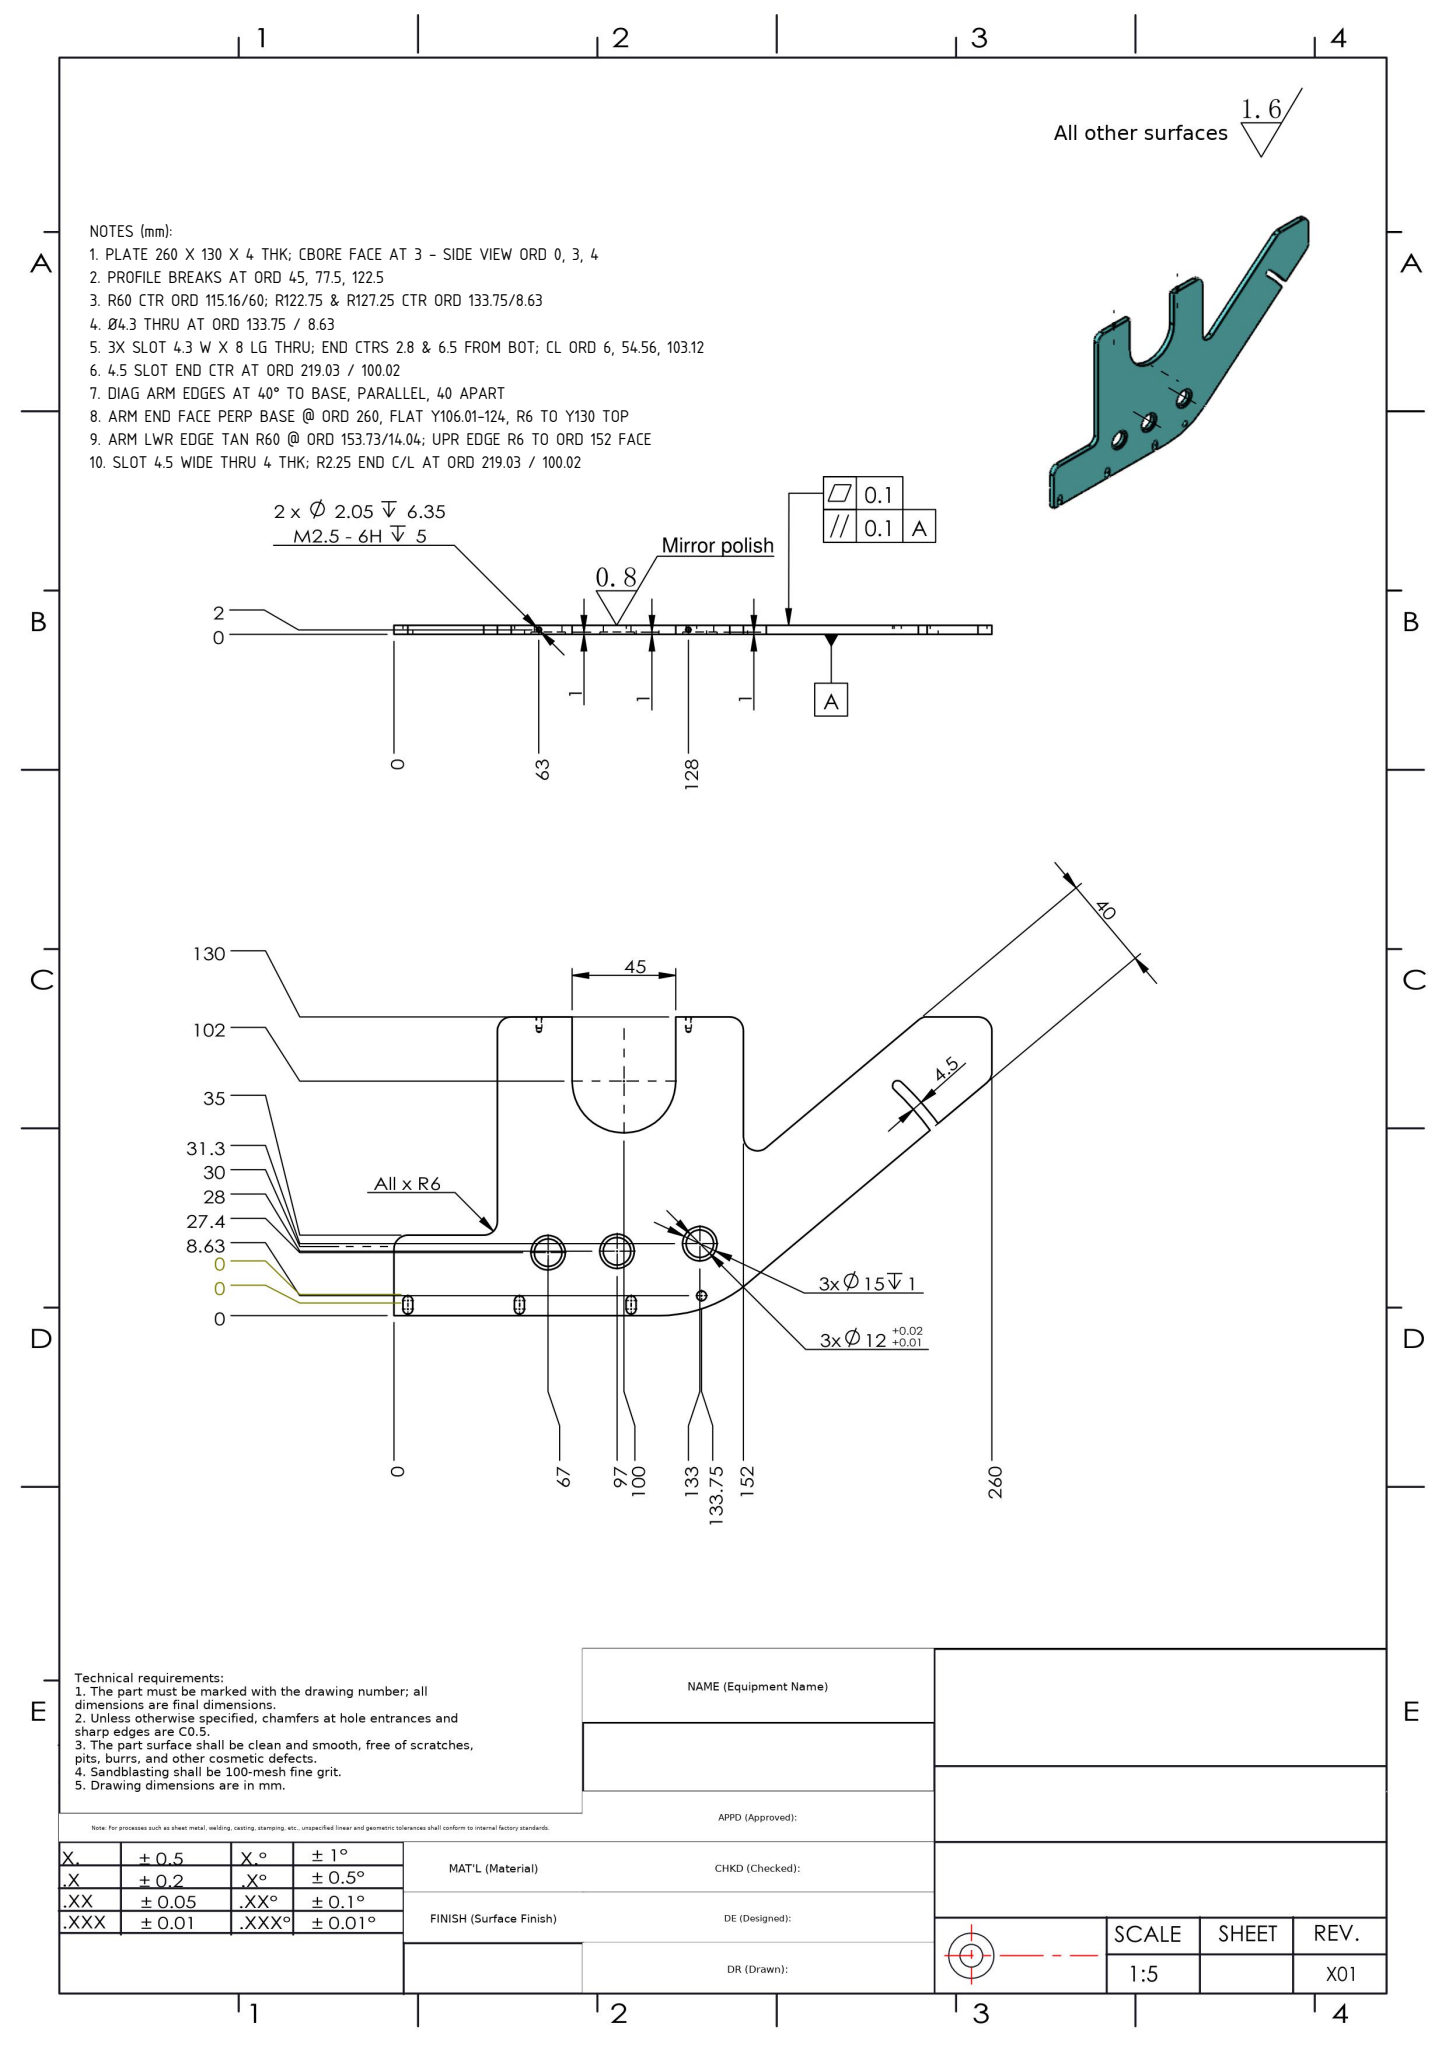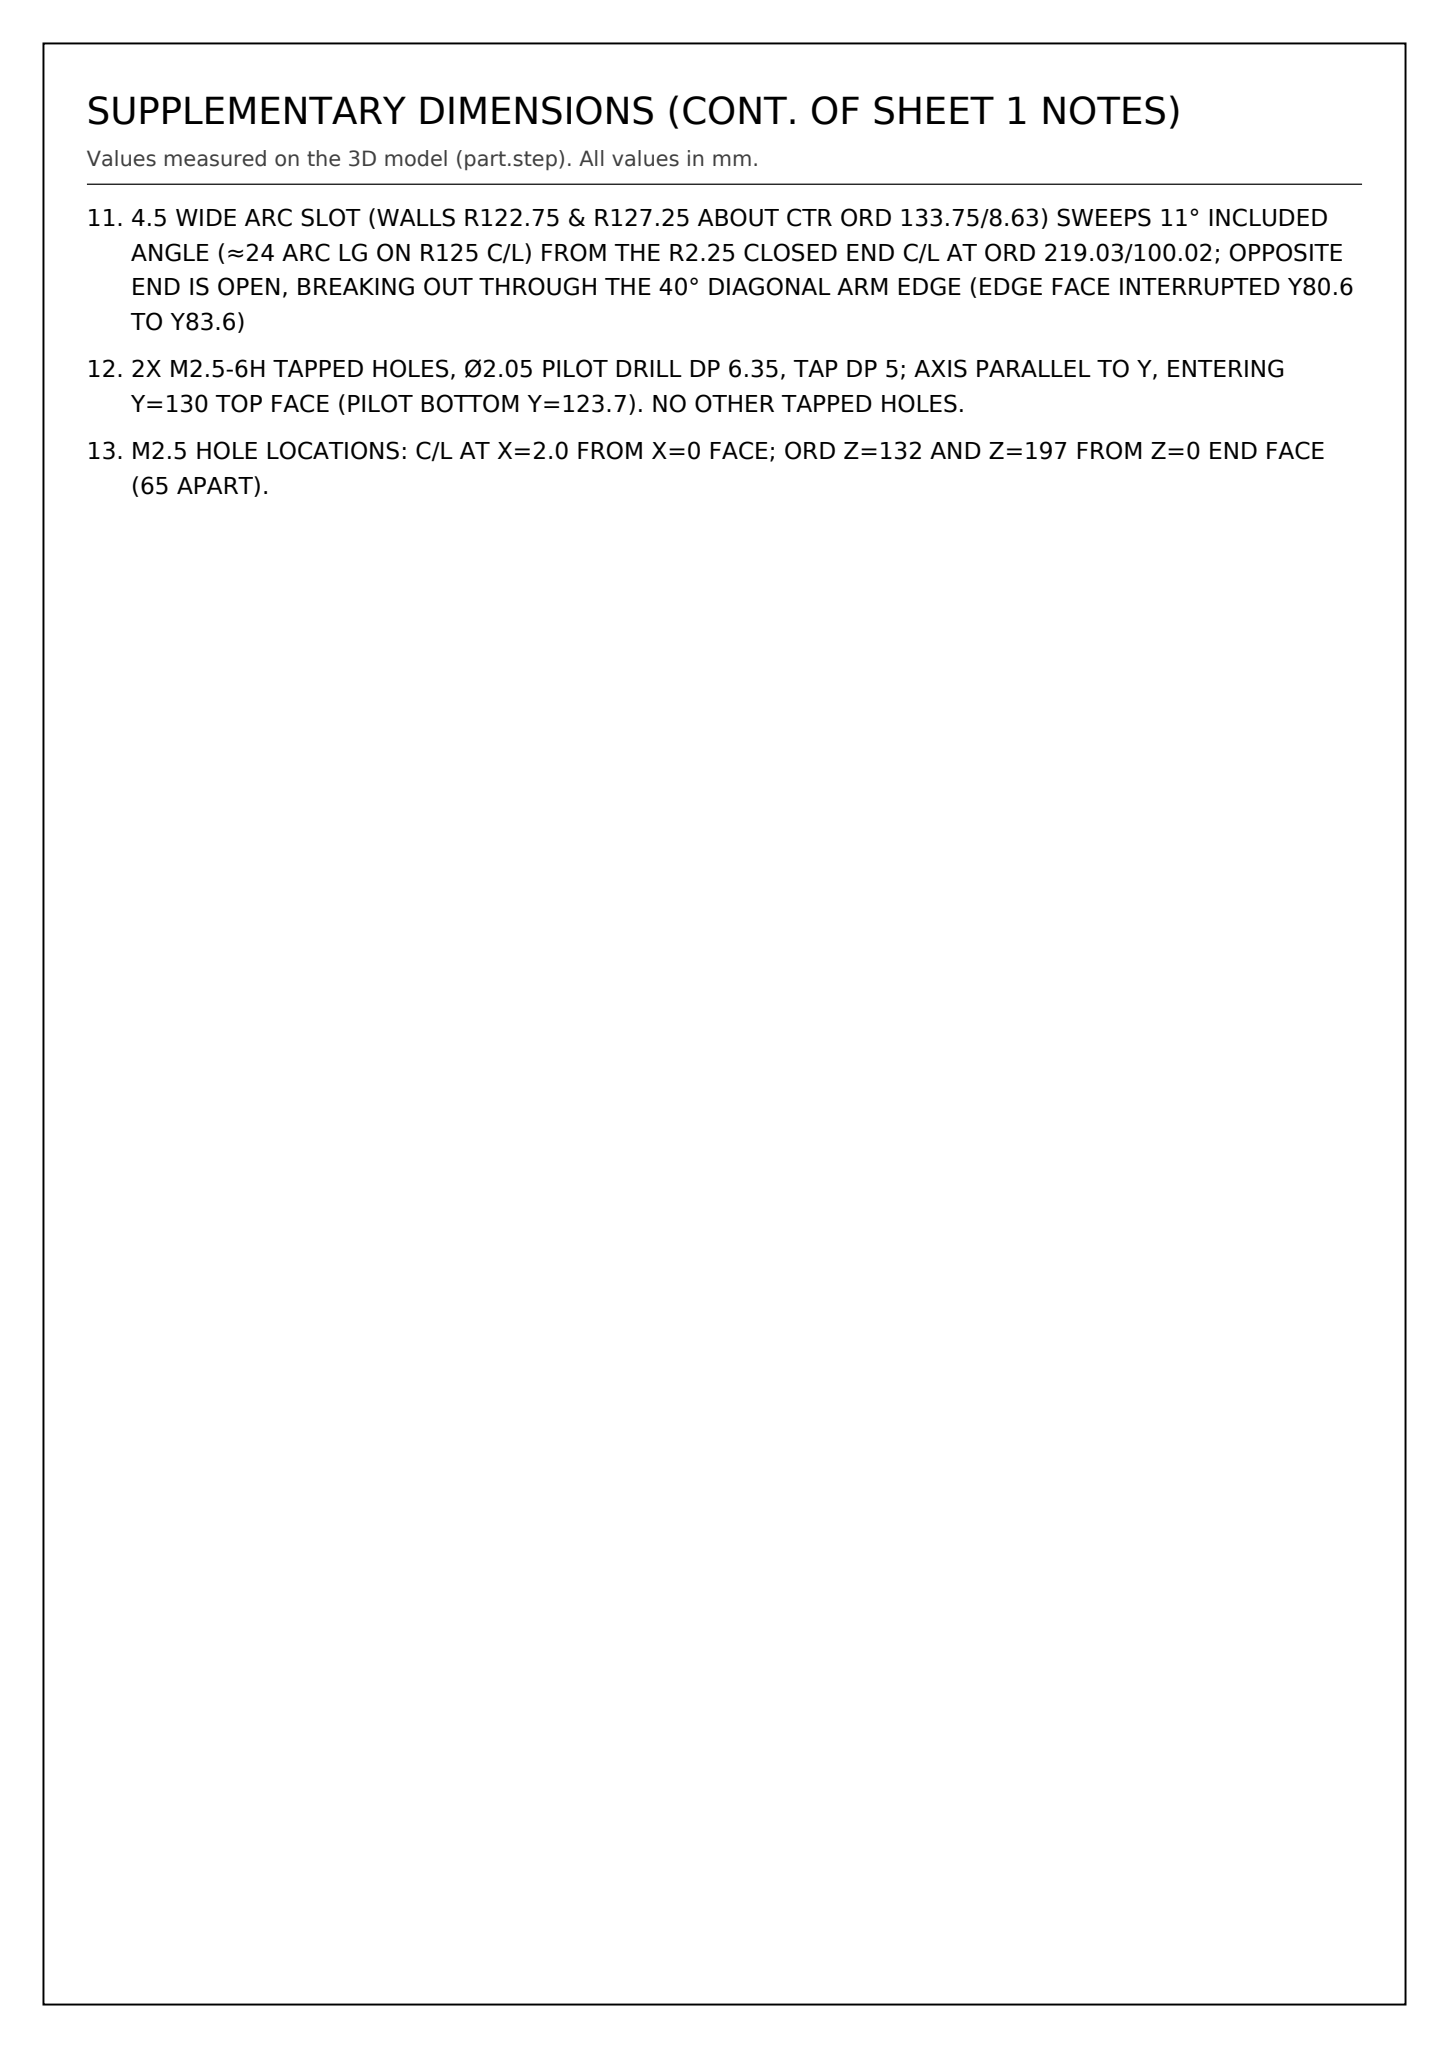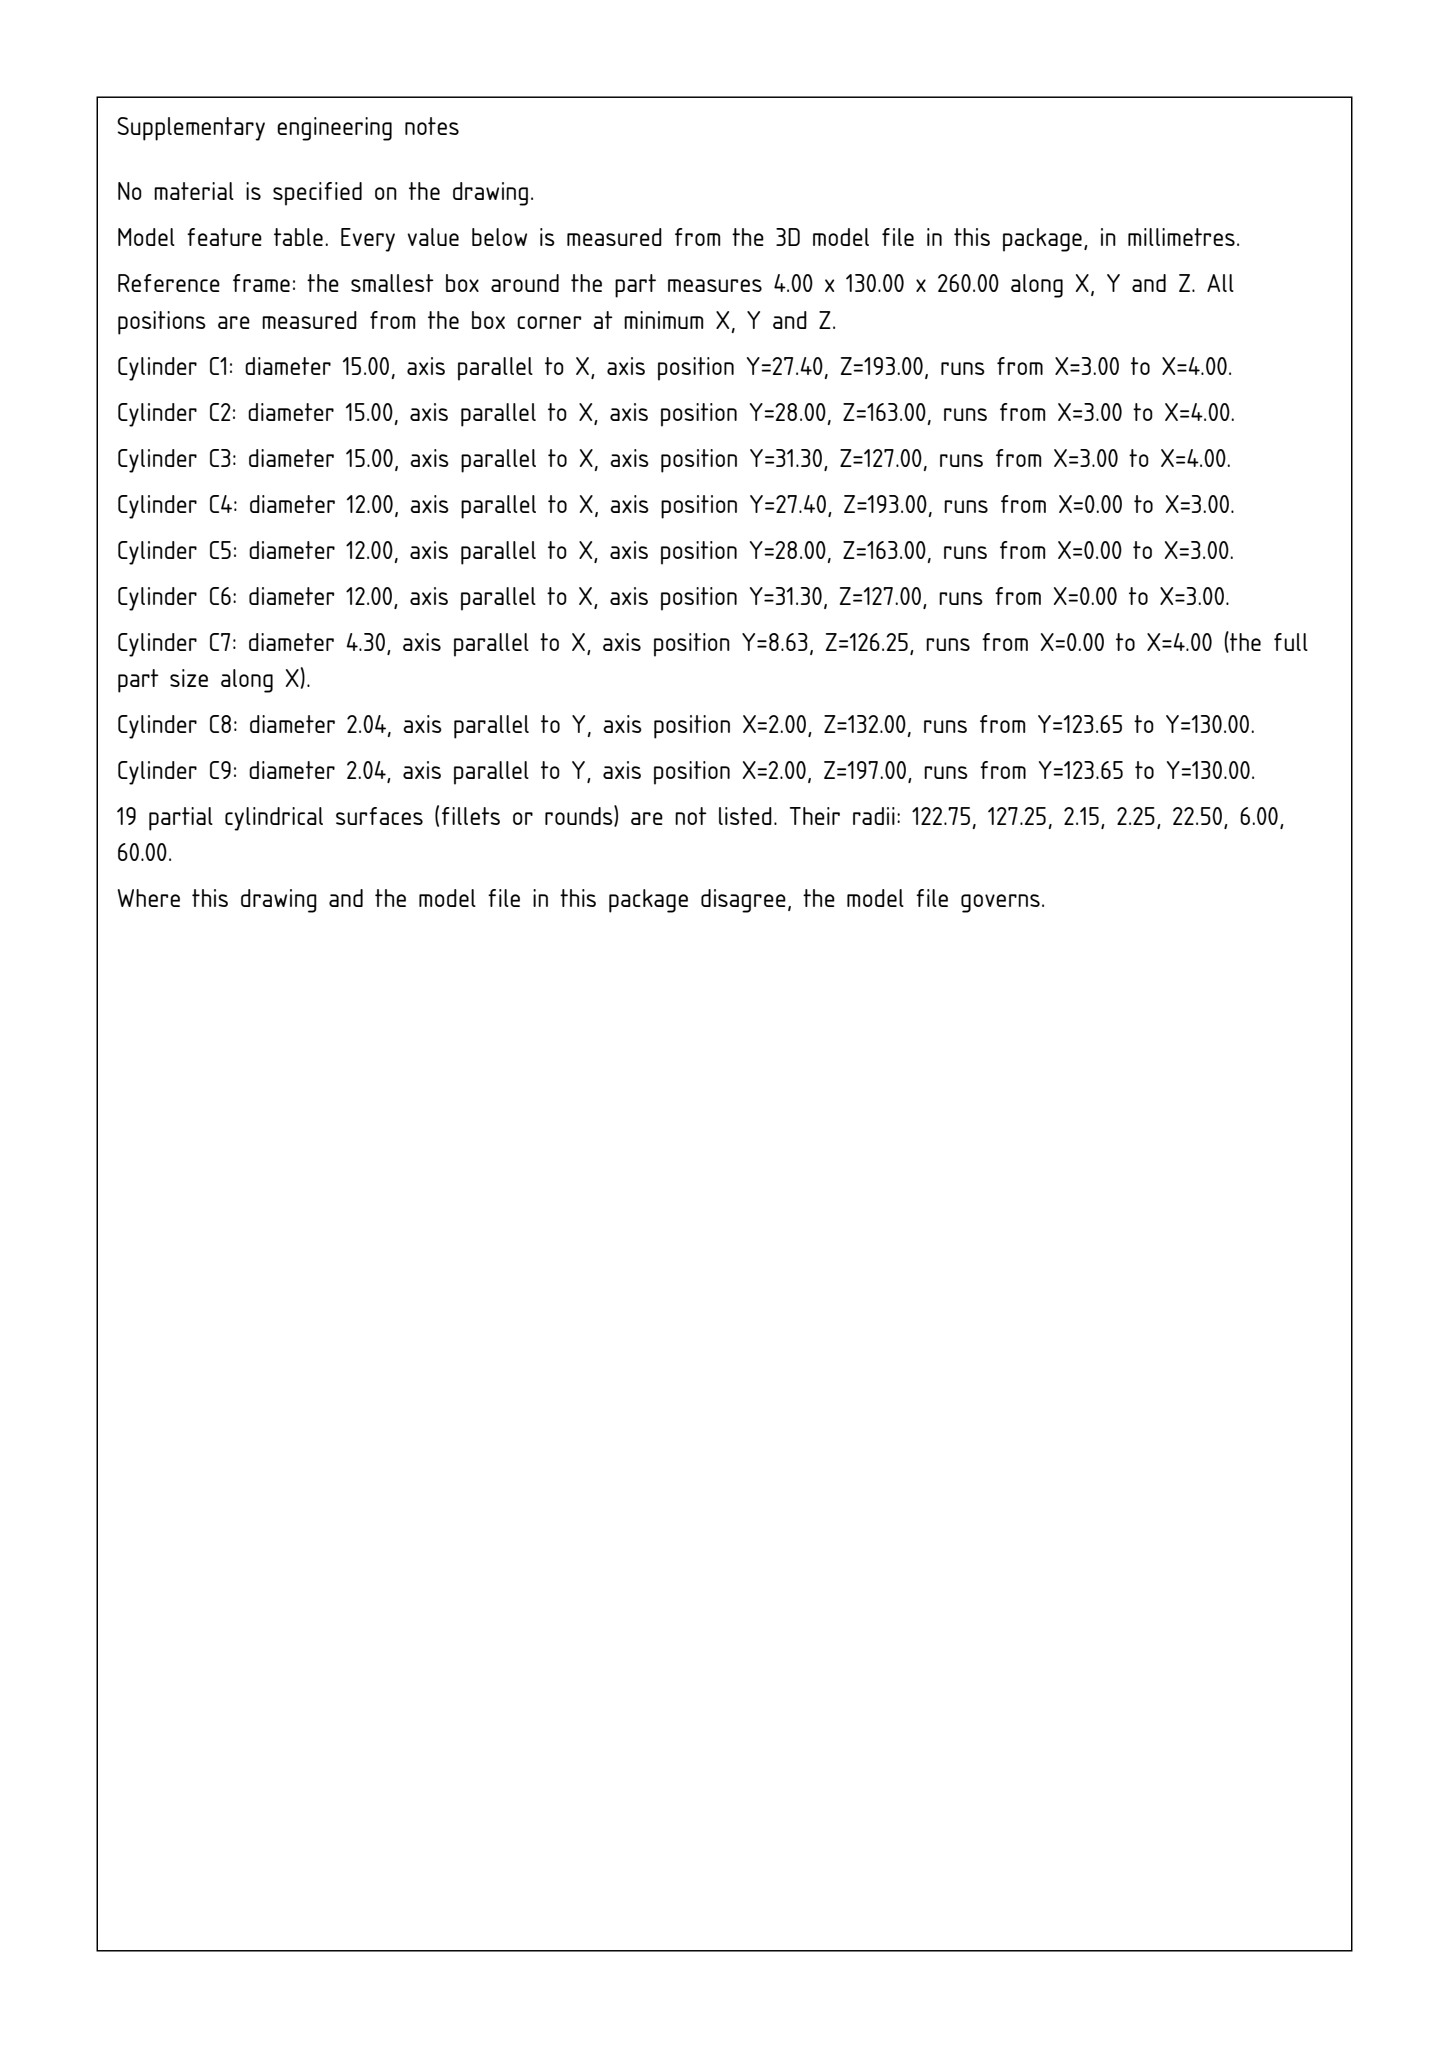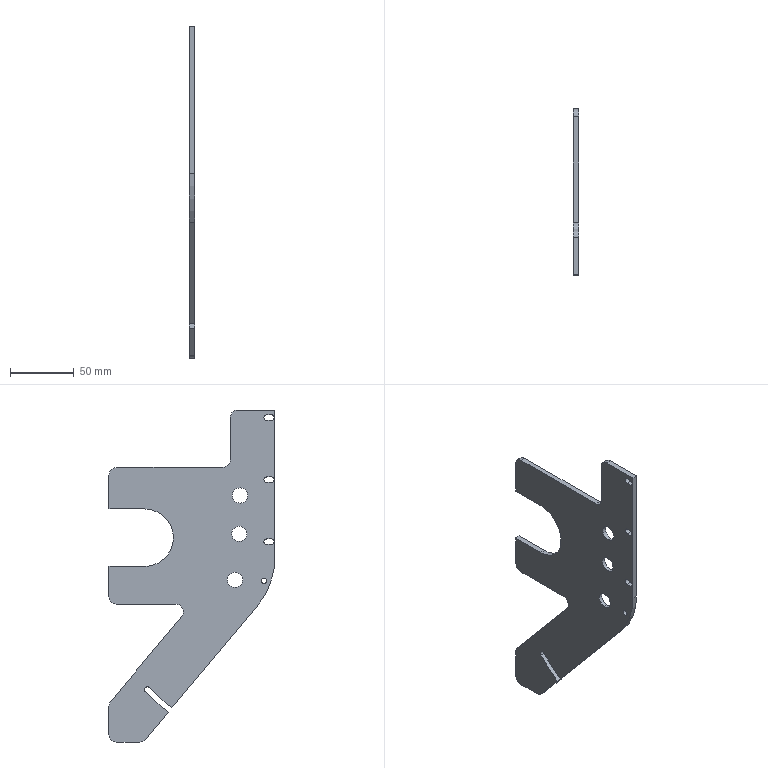Part | SolidWorks | mm | 1 solid | 66 faces | box 4 x 130 x 260 mm | volume 71713 mm3 | cylinder 37 | plane 25 | cone 4 | commonest cylinder face diameters 12 x14 4.3 x8 15 x6 2.05 x4 120 x1 245.5 x1 254.5 x1 4.5 x1
Drawing notes:
PLATE 260 X 130 X 4 THK; CBORE FACE AT 3 - SIDE VIEW ORD 0, 3, 4 | from the solid: bbox_xyz [4,130,260]; axis_planes x=0.0, 3.0 (3), 4.0
PROFILE BREAKS AT ORD 45, 77.5, 122.5 | from the solid: axis_planes z=215, 182.5, 137.5; ord = 260 - z
R60 CTR ORD 115.16/60; R122.75 & R127.25 CTR ORD 133.75/8.63 | from the solid: Ø120 at [y=60,z=144.84]; Ø245.5 & Ø254.5 at [y=8.63,z=126.25]
Ø4.3 THRU AT ORD 133.75 / 8.63 | from the solid: [4.3,"x",[null,8.63,126.25],4.0]; ord = 260-126.25 = 133.75
3X SLOT 4.3 W X 8 LG THRU; END CTRS 2.8 & 6.5 FROM BOT; CL ORD 6, 54.56, 103.12 | from the solid: Ø4.3 x-axis cyls at y=2.8 & 6.5, len 4.0 thru, z=156.88/205.44/254.0; 6.5-2.8+4.3=8; ord = 260-z
4.5 SLOT END CTR AT ORD 219.03 / 100.02 | from the solid: [4.5,"x",[null,100.02,40.97],4.0]; ord = 260-40.97 = 219.03
DIAG ARM EDGES AT 40° TO BASE, PARALLEL, 40 APART | from the solid: Upper edge tangent to R6 fillet ctr (ORD 231.88,Y124), lower edge tangent to R6 fillet ctr (ORD 254,Y106.01); common normal gives 40.0° to ORD axis and 40.00 perpendicular spacing (matches 40 width dim)
ARM END FACE PERP BASE @ ORD 260, FLAT Y106.01-124, R6 TO Y130 TOP | from the solid: Planar face normal z at z=0 (ORD 260 = 260-z); R6 (Ø12) fillet ctrs at y=106.01/z=6 and y=124/z=6; plane y=130 top face tangent to R6 ctr y=124, z=28.12 (ORD 231.88-254)
ARM LWR EDGE TAN R60 @ ORD 153.73/14.04; UPR EDGE R6 TO ORD 152 FACE | from the solid: Ø120 (R60) cyl ctr y=60,z=144.84 (ORD 115.16); dist from ctr to lower edge line = 59.99; R6 fillet ctr y=77.67,z=102 (ORD 158) tangent to upper edge and to plane z=108 (ORD 152)
SLOT 4.5 WIDE THRU 4 THK; R2.25 END C/L AT ORD 219.03 / 100.02 | from the solid: cylinders: [4.5,"x",[null,100.02,40.97],4.0,1]; bbox z=260 so ORD = 260-40.97 = 219.03; plate thk 4 (x planes 0.0 and 4.0)
4.5 WIDE ARC SLOT (WALLS R122.75 & R127.25 ABOUT CTR ORD 133.75/8.63) SWEEPS 11° INCLUDED ANGLE (≈24 ARC LG ON R125 C/L) FROM THE R2.25 CLOSED END C/L AT ORD 219.03/100.02; OPPOSITE END IS OPEN, BREAKING OUT THROUGH THE 40° DIAGONAL ARM EDGE (EDGE FACE INTERRUPTED Y80.6 TO Y83.6) | from the solid: cylinders: concave arc dia 254.5 and convex arc dia 245.5, axis x, centre (y 8.6, z 126.3), from 0 to 4, arc_deg 11 (= R127.25/R122.75 slot walls about ORD 133.75/8.63); concave arc dia 4.5 at (y 100.0, z 41.0) thru 0-4 = closed end; inclined_planes at 40°: bbox_from [0,14,26.9] size [4,66.6,79.4] and bbox_from [0,83.6,2.1] size [4,17.8,21.3] are collinear arm-edge faces separated by the slot breakout
2X M2.5-6H TAPPED HOLES, Ø2.05 PILOT DRILL DP 6.35, TAP DP 5; AXIS PARALLEL TO Y, ENTERING Y=130 TOP FACE (PILOT BOTTOM Y=123.7). NO OTHER TAPPED HOLES. | from the solid: cylinders: only two 'hole/bore' Ø2.05 with axis y, from y=123.7 to y=130.0
M2.5 HOLE LOCATIONS: C/L AT X=2.0 FROM X=0 FACE; ORD Z=132 AND Z=197 FROM Z=0 END FACE (65 APART). | from the solid: cylinders: Ø2.05 axis y at axis_pos (x=2.0, z=132.0) and (x=2.0, z=197.0)